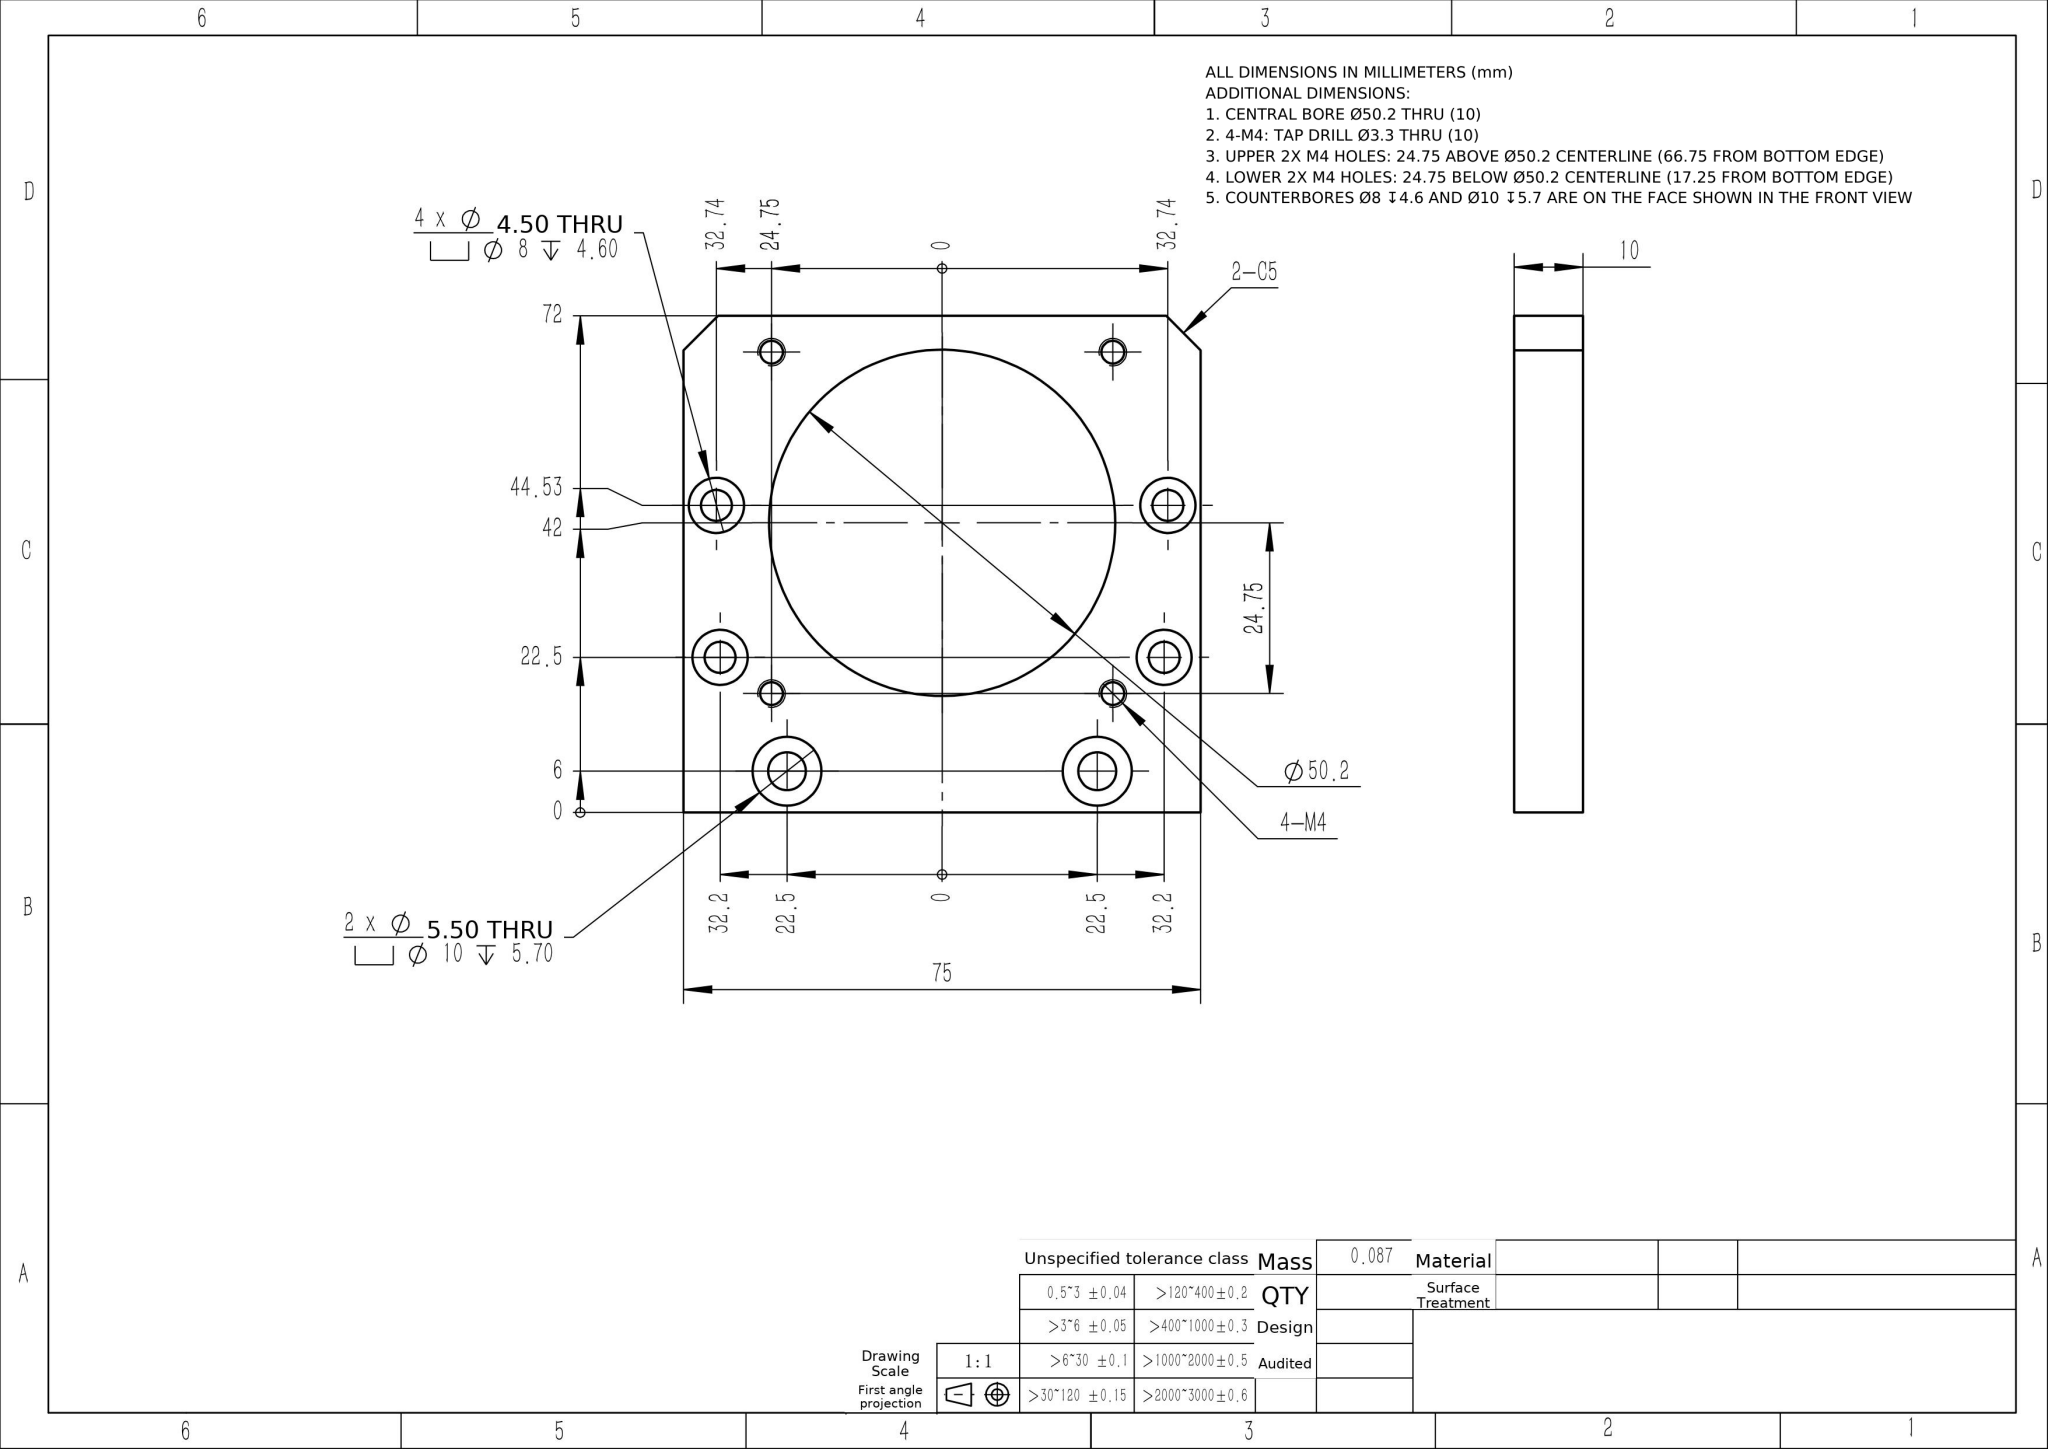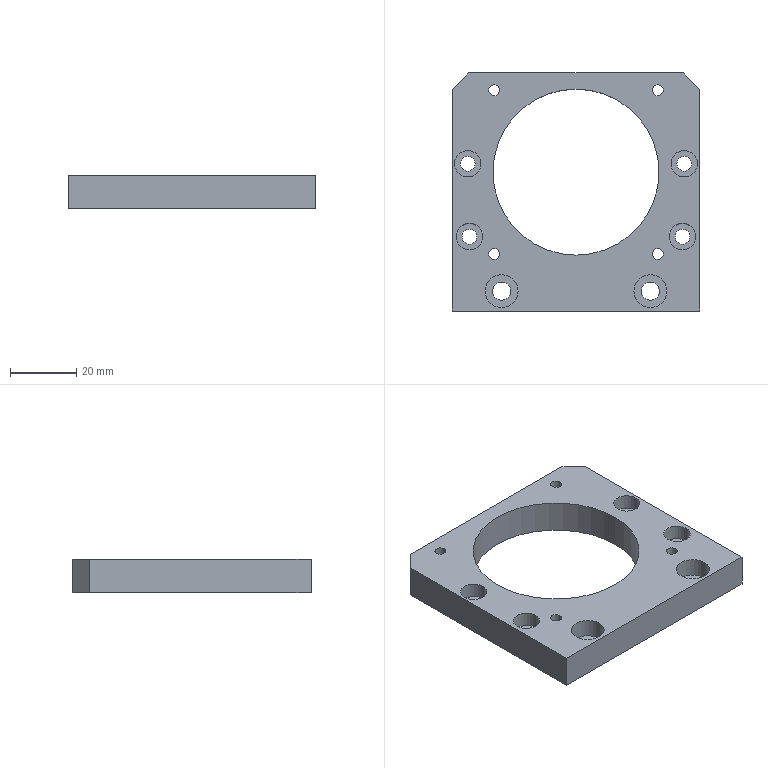Part | NX | mm | 1 solid | 48 faces | box 75 x 72 x 10 mm | volume 31247 mm3 | cylinder 34 | plane 14 | commonest cylinder face diameters 8 x8 4.5 x8 3.3 x8 10 x4 5.5 x4 50.2 x2